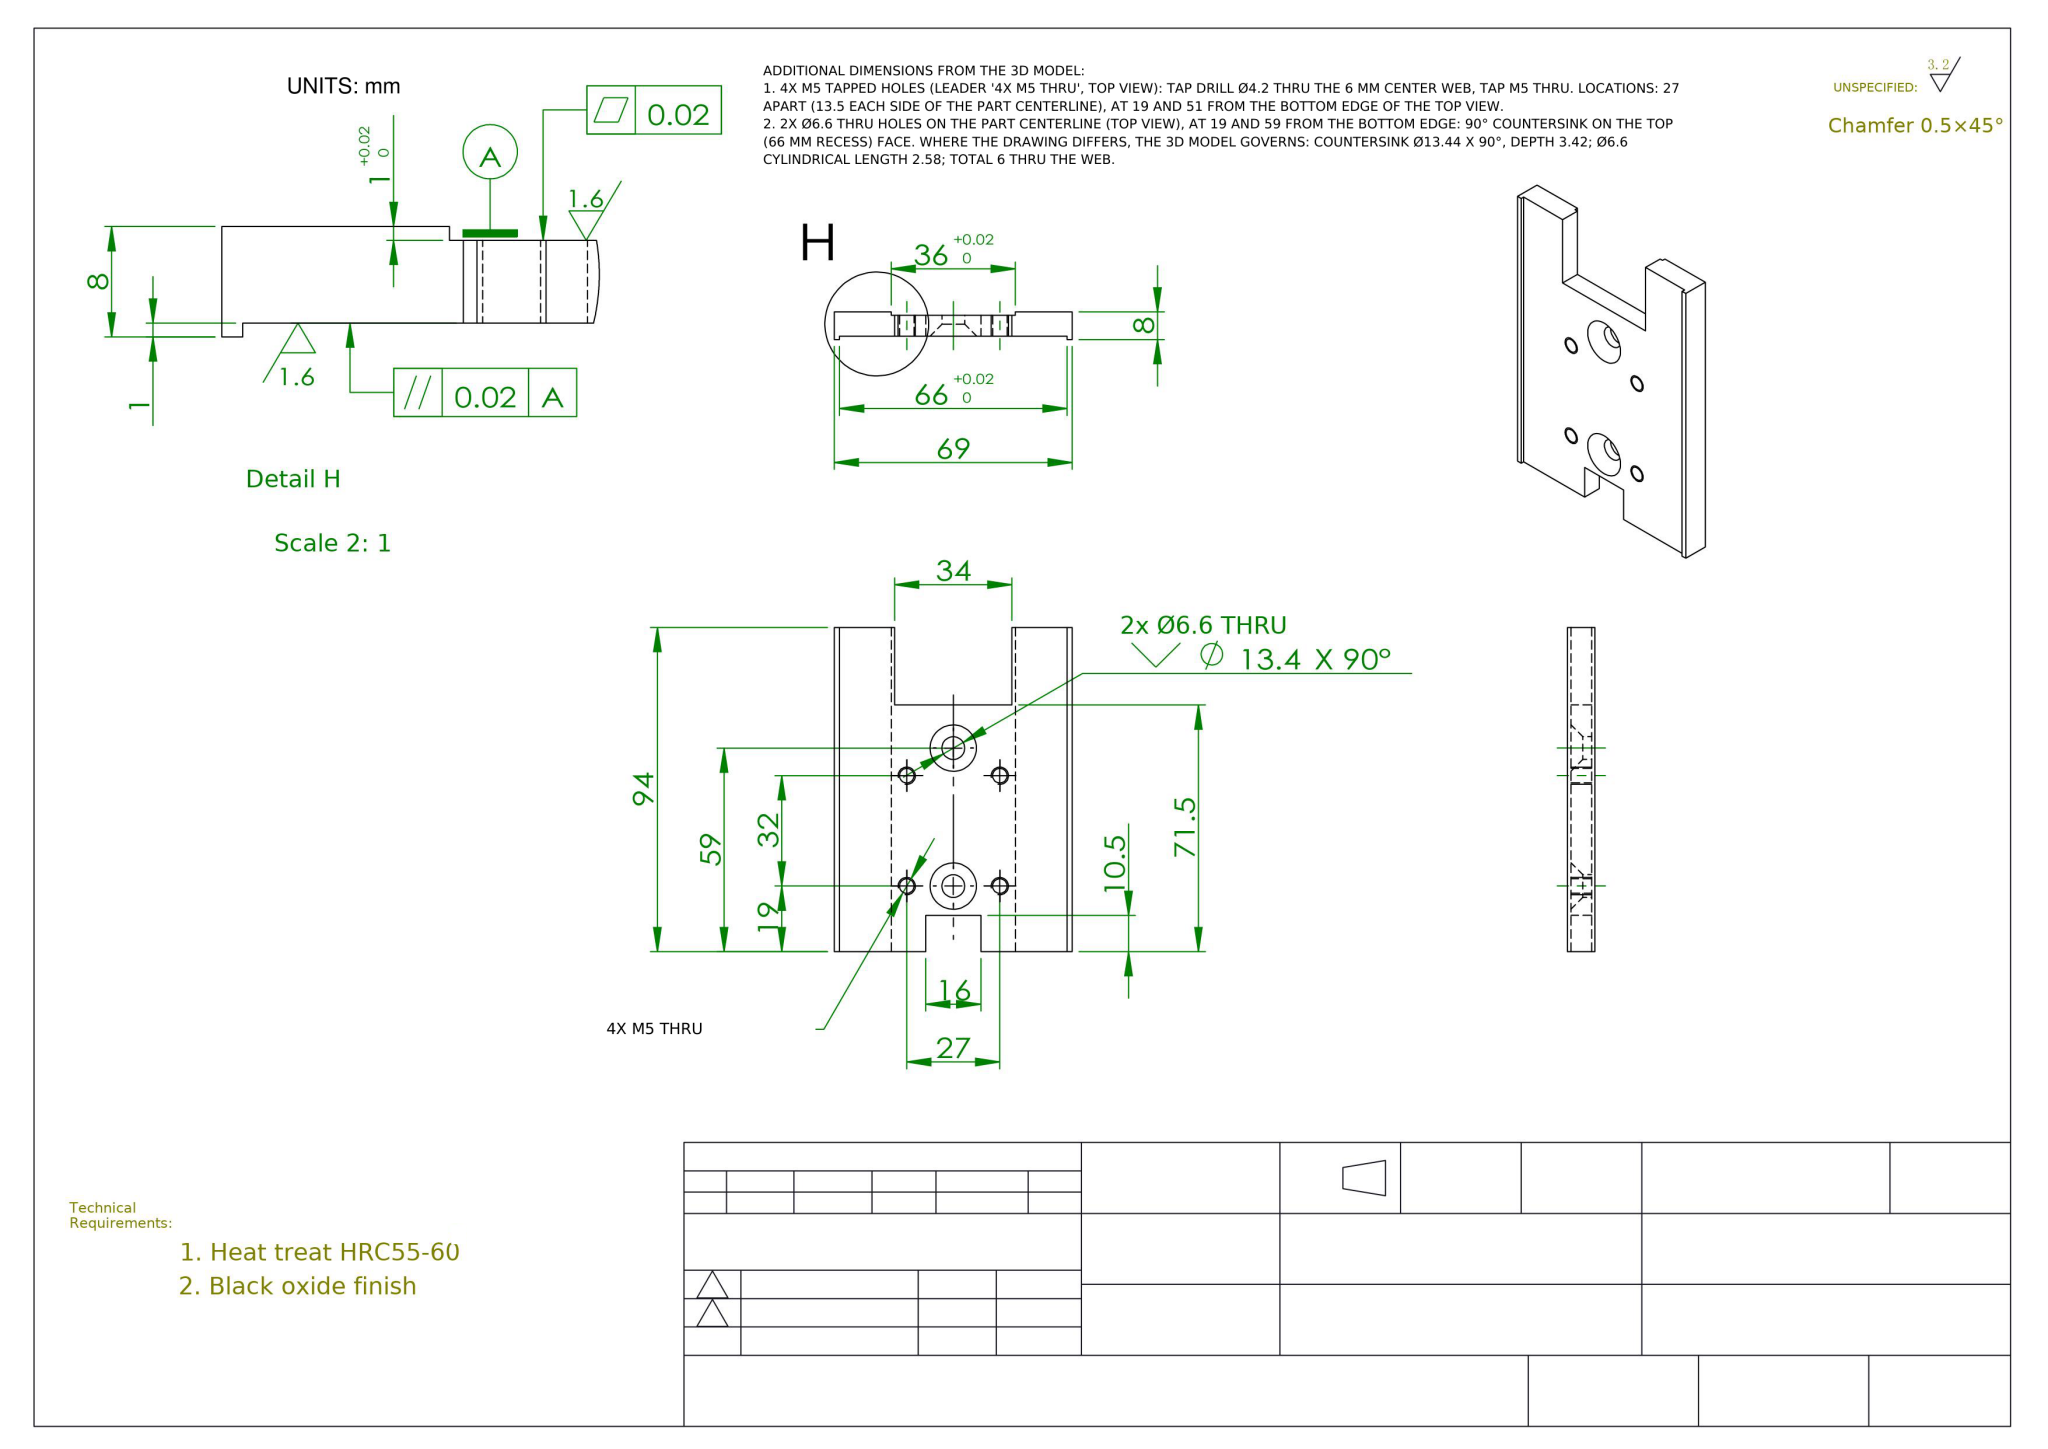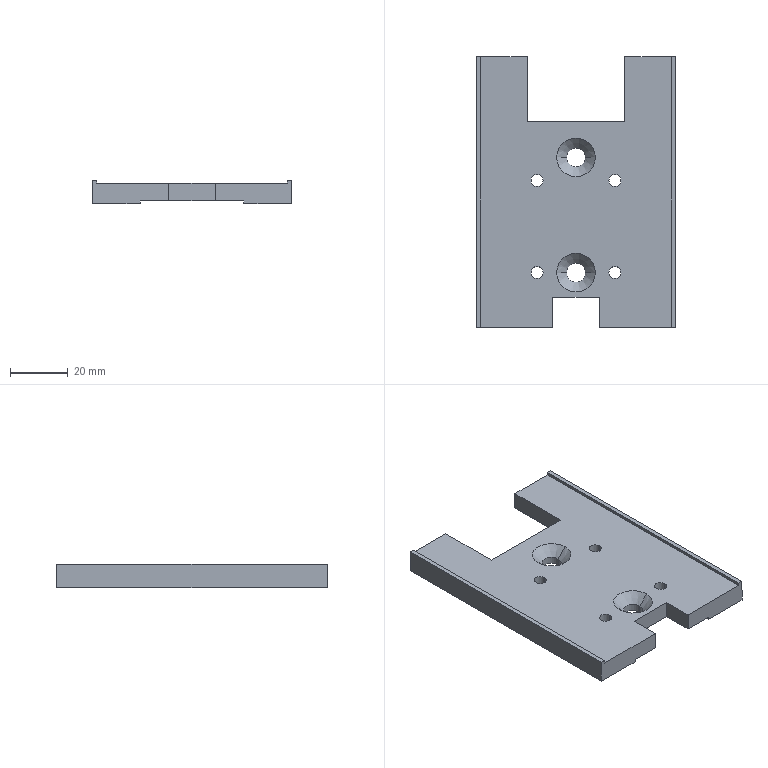Part | NX | mm | 1 solid | 38 faces | box 69 x 94 x 8 mm | volume 35633 mm3 | plane 22 | cylinder 12 | cone 4 | commonest cylinder face diameters 4.2 x8 6.6 x4